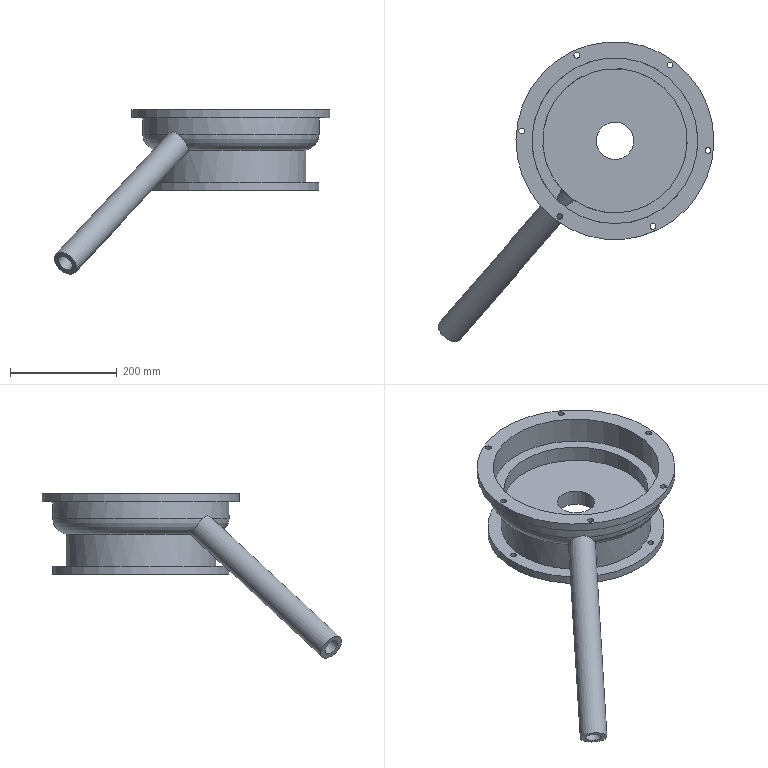Component | NX | GEARBOX | 1 solid | 31 faces | volume 4100107 mm3 | cylinder 22 | plane 8 | torus 1 | commonest cylinder face diameters 11 x12 270 x2 330 x2 30 x1 50 x1 370 x1 310 x1 280 x1